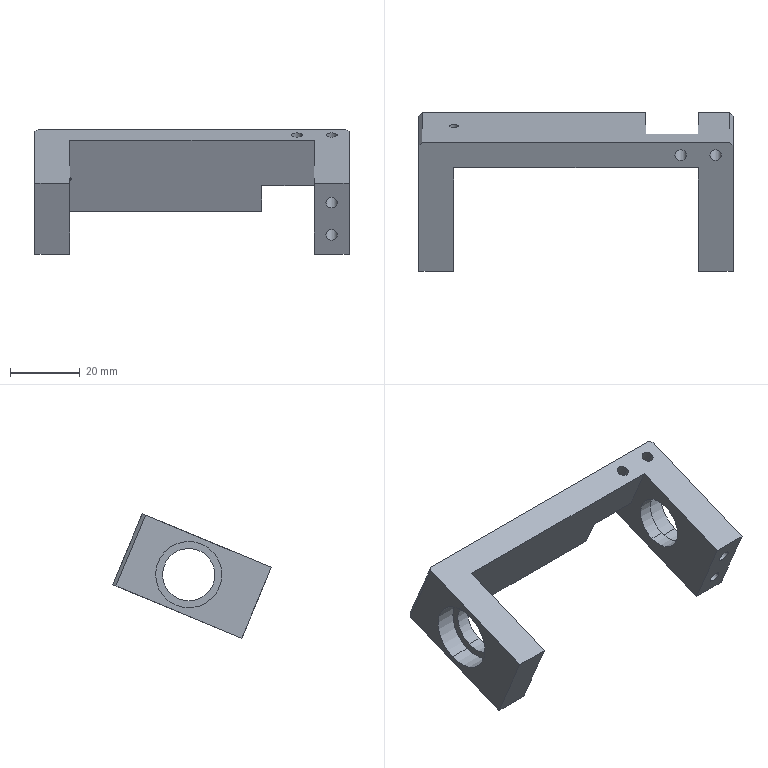Component | SolidWorks | 04-007BearingHousing-4 | 1 solid | 44 faces | volume 23252 mm3 | cylinder 18 | plane 17 | cone 9 | commonest cylinder face diameters 3.3 x8 19 x4 15 x4 2.5 x2